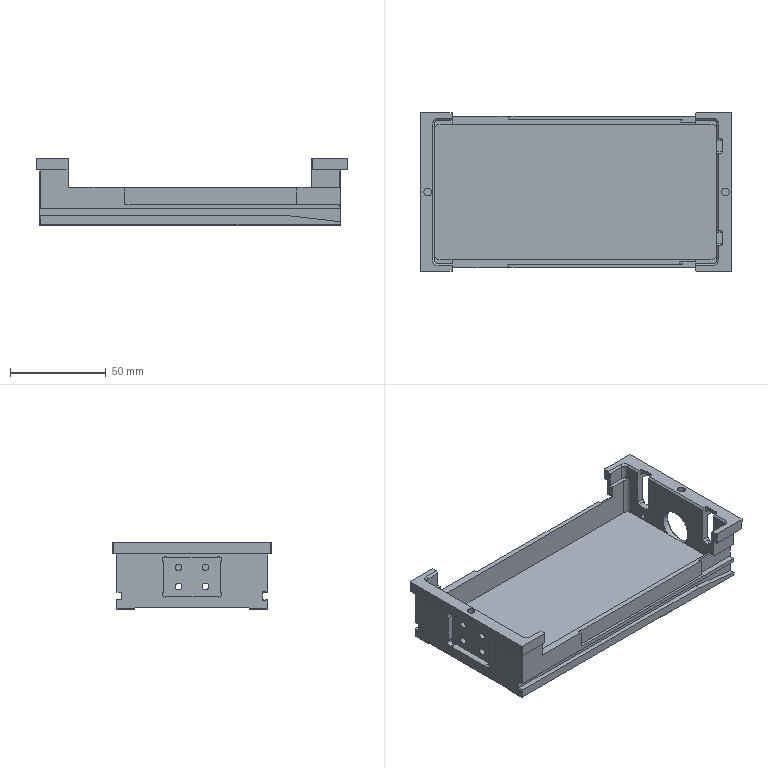CAM job | NX | mm | 3-axis | 1 set-up | 4 operations | part box 163 x 83 x 35
set-up 1
1. Cavity Milling | Mill Mill5 D10 | CAVITY_MILL | path 1919.089 mm | 7.253 min
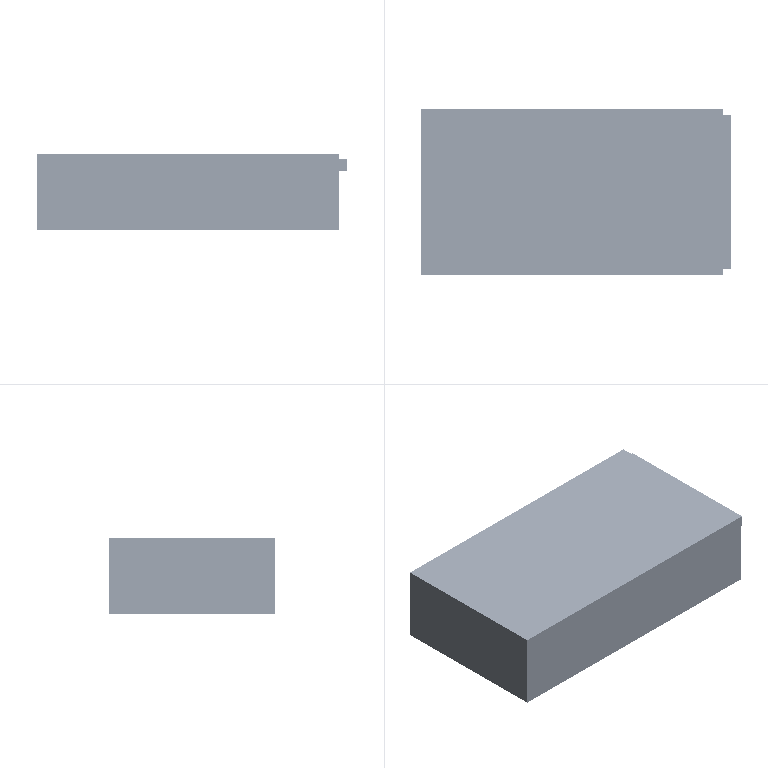2. Volume Based 2.5D Milling | Mill Mill5 D4 | FLOOR_WALL | path 1462.328 mm | 5.005 min
3. Cavity Milling | Mill Mill5 D4 | CAVITY_MILL_1 | path 3745.65 mm | 10.984 min
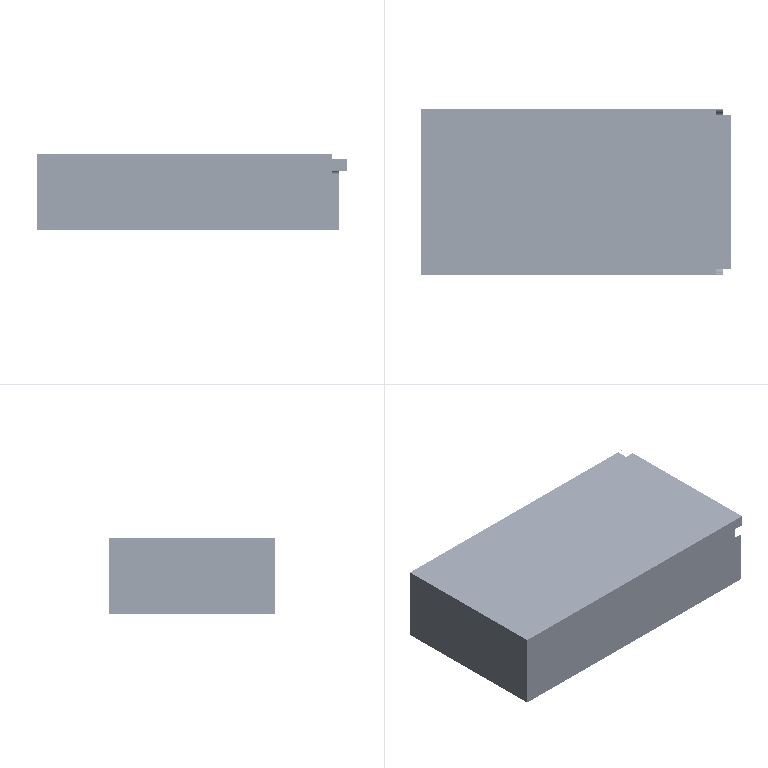4. Planar Milling | Mill Mill5 D4 | PLANAR_PROFILE | path 106.03 mm | 0.3149 min